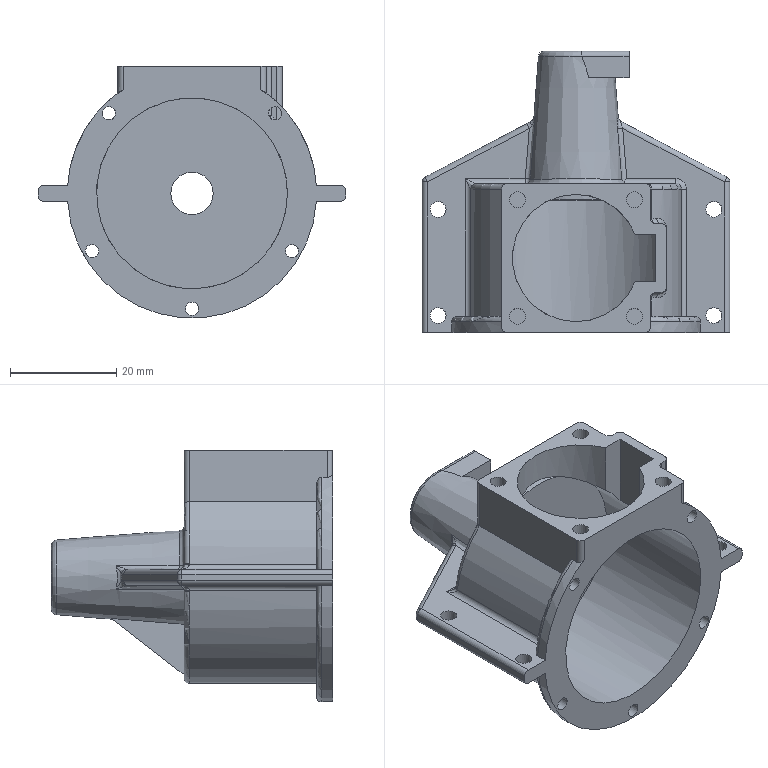Component | NX | CYLINDER_BLOCK | 1 solid | 131 faces | volume 18201 mm3 | cylinder 54 | plane 39 | spline 19 | torus 11 | sphere 7 | cone 1 | commonest cylinder face diameters 2 x31 3 x8 2.5 x5 47 x3 40 x3 36 x2 8 x1 24 x1